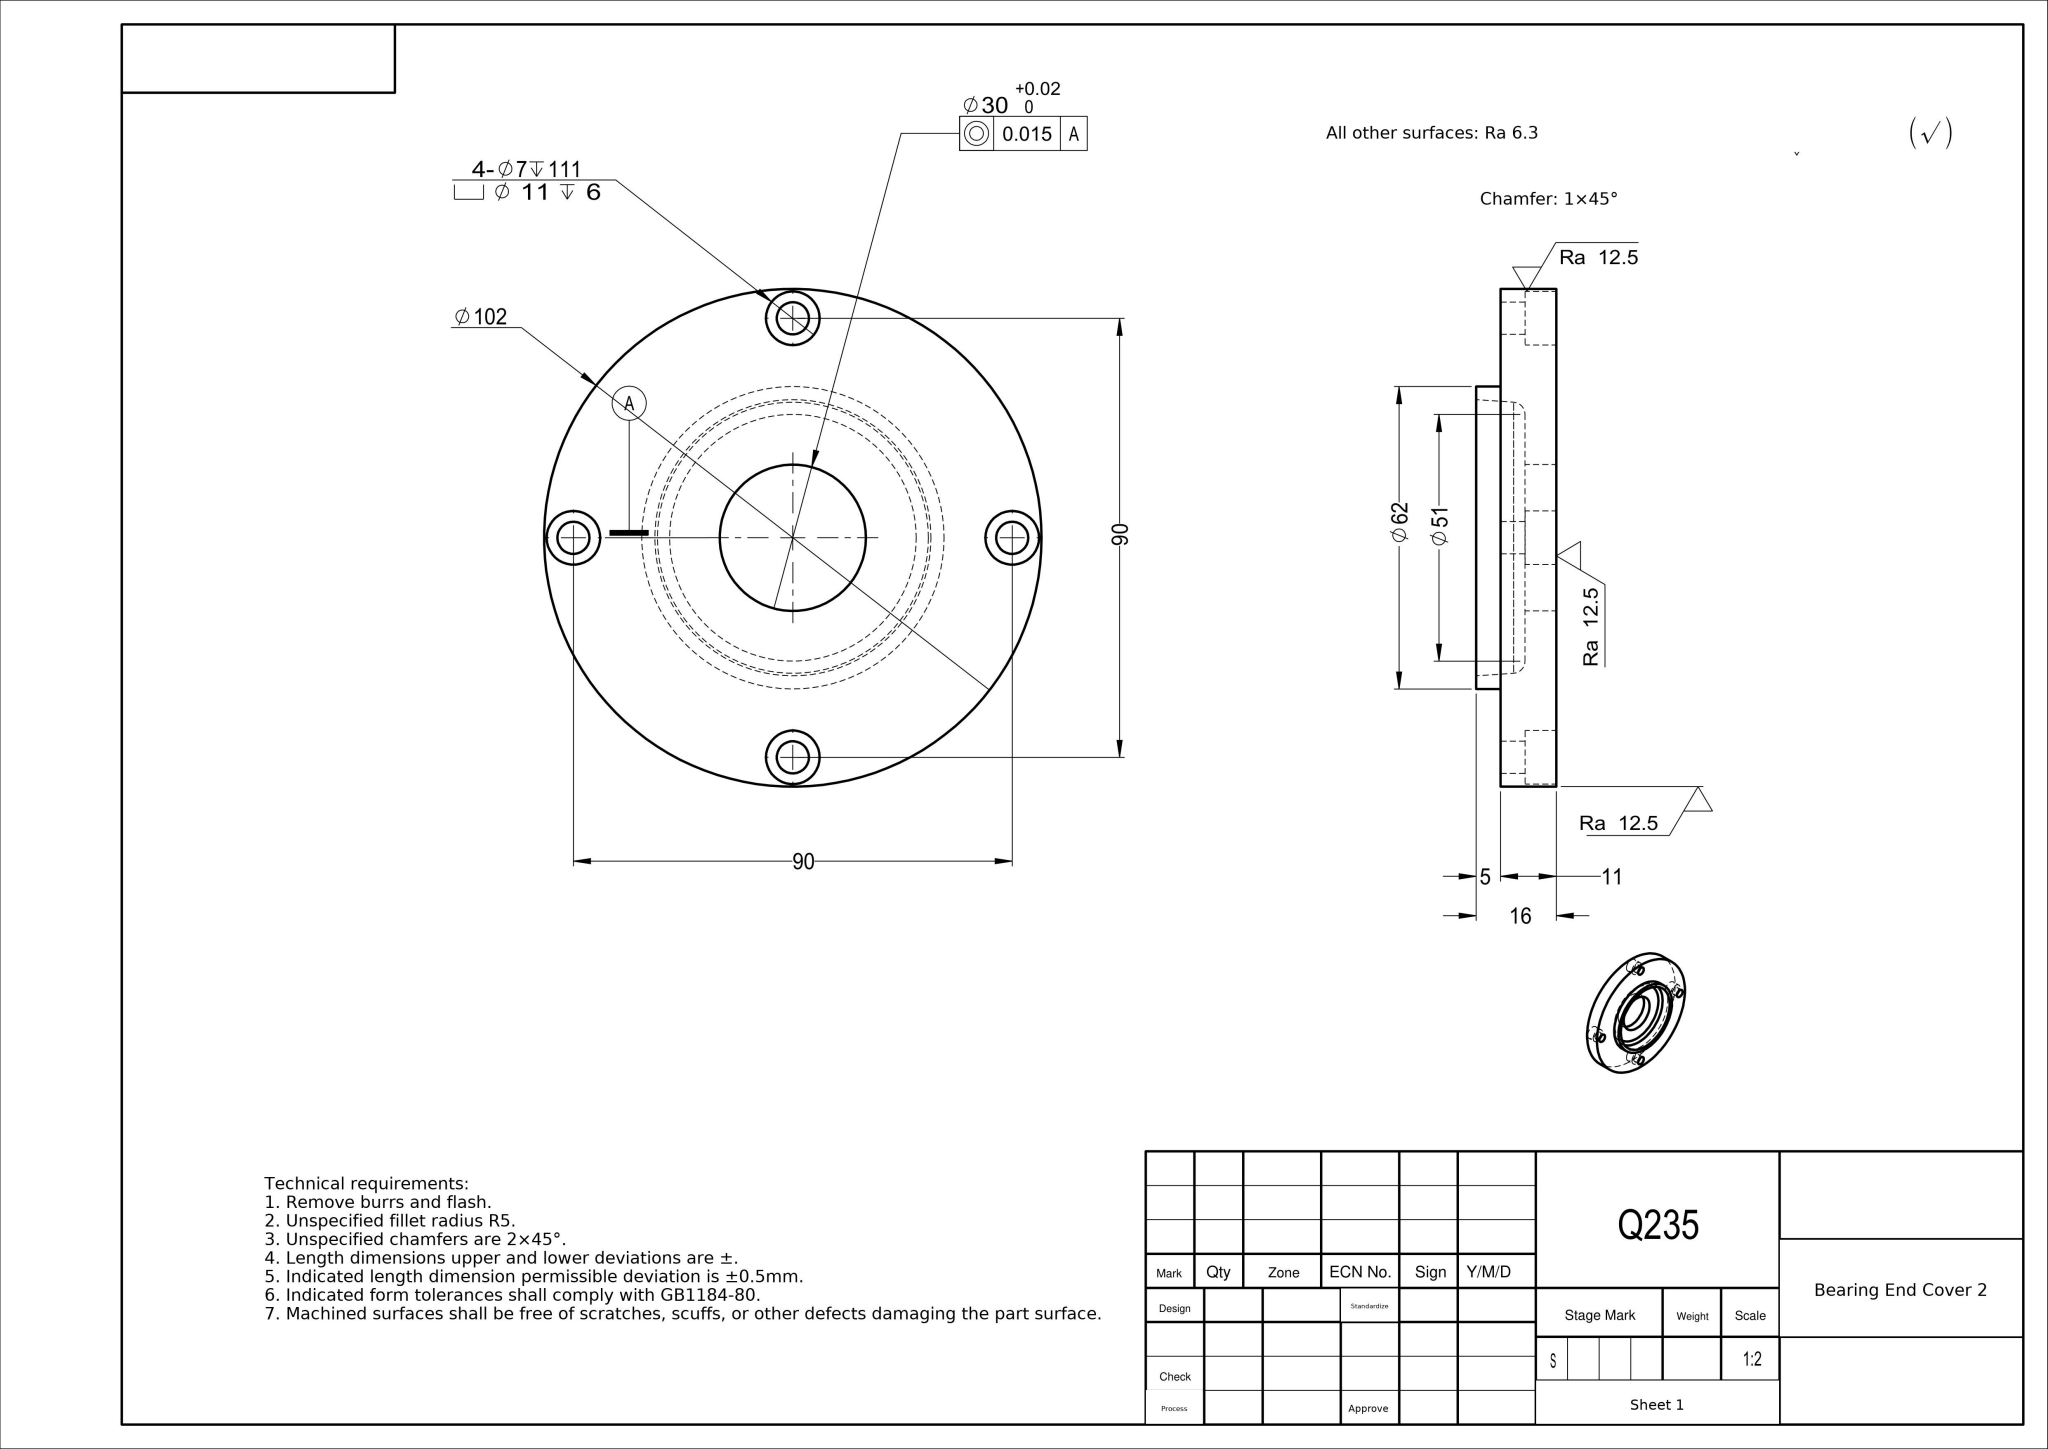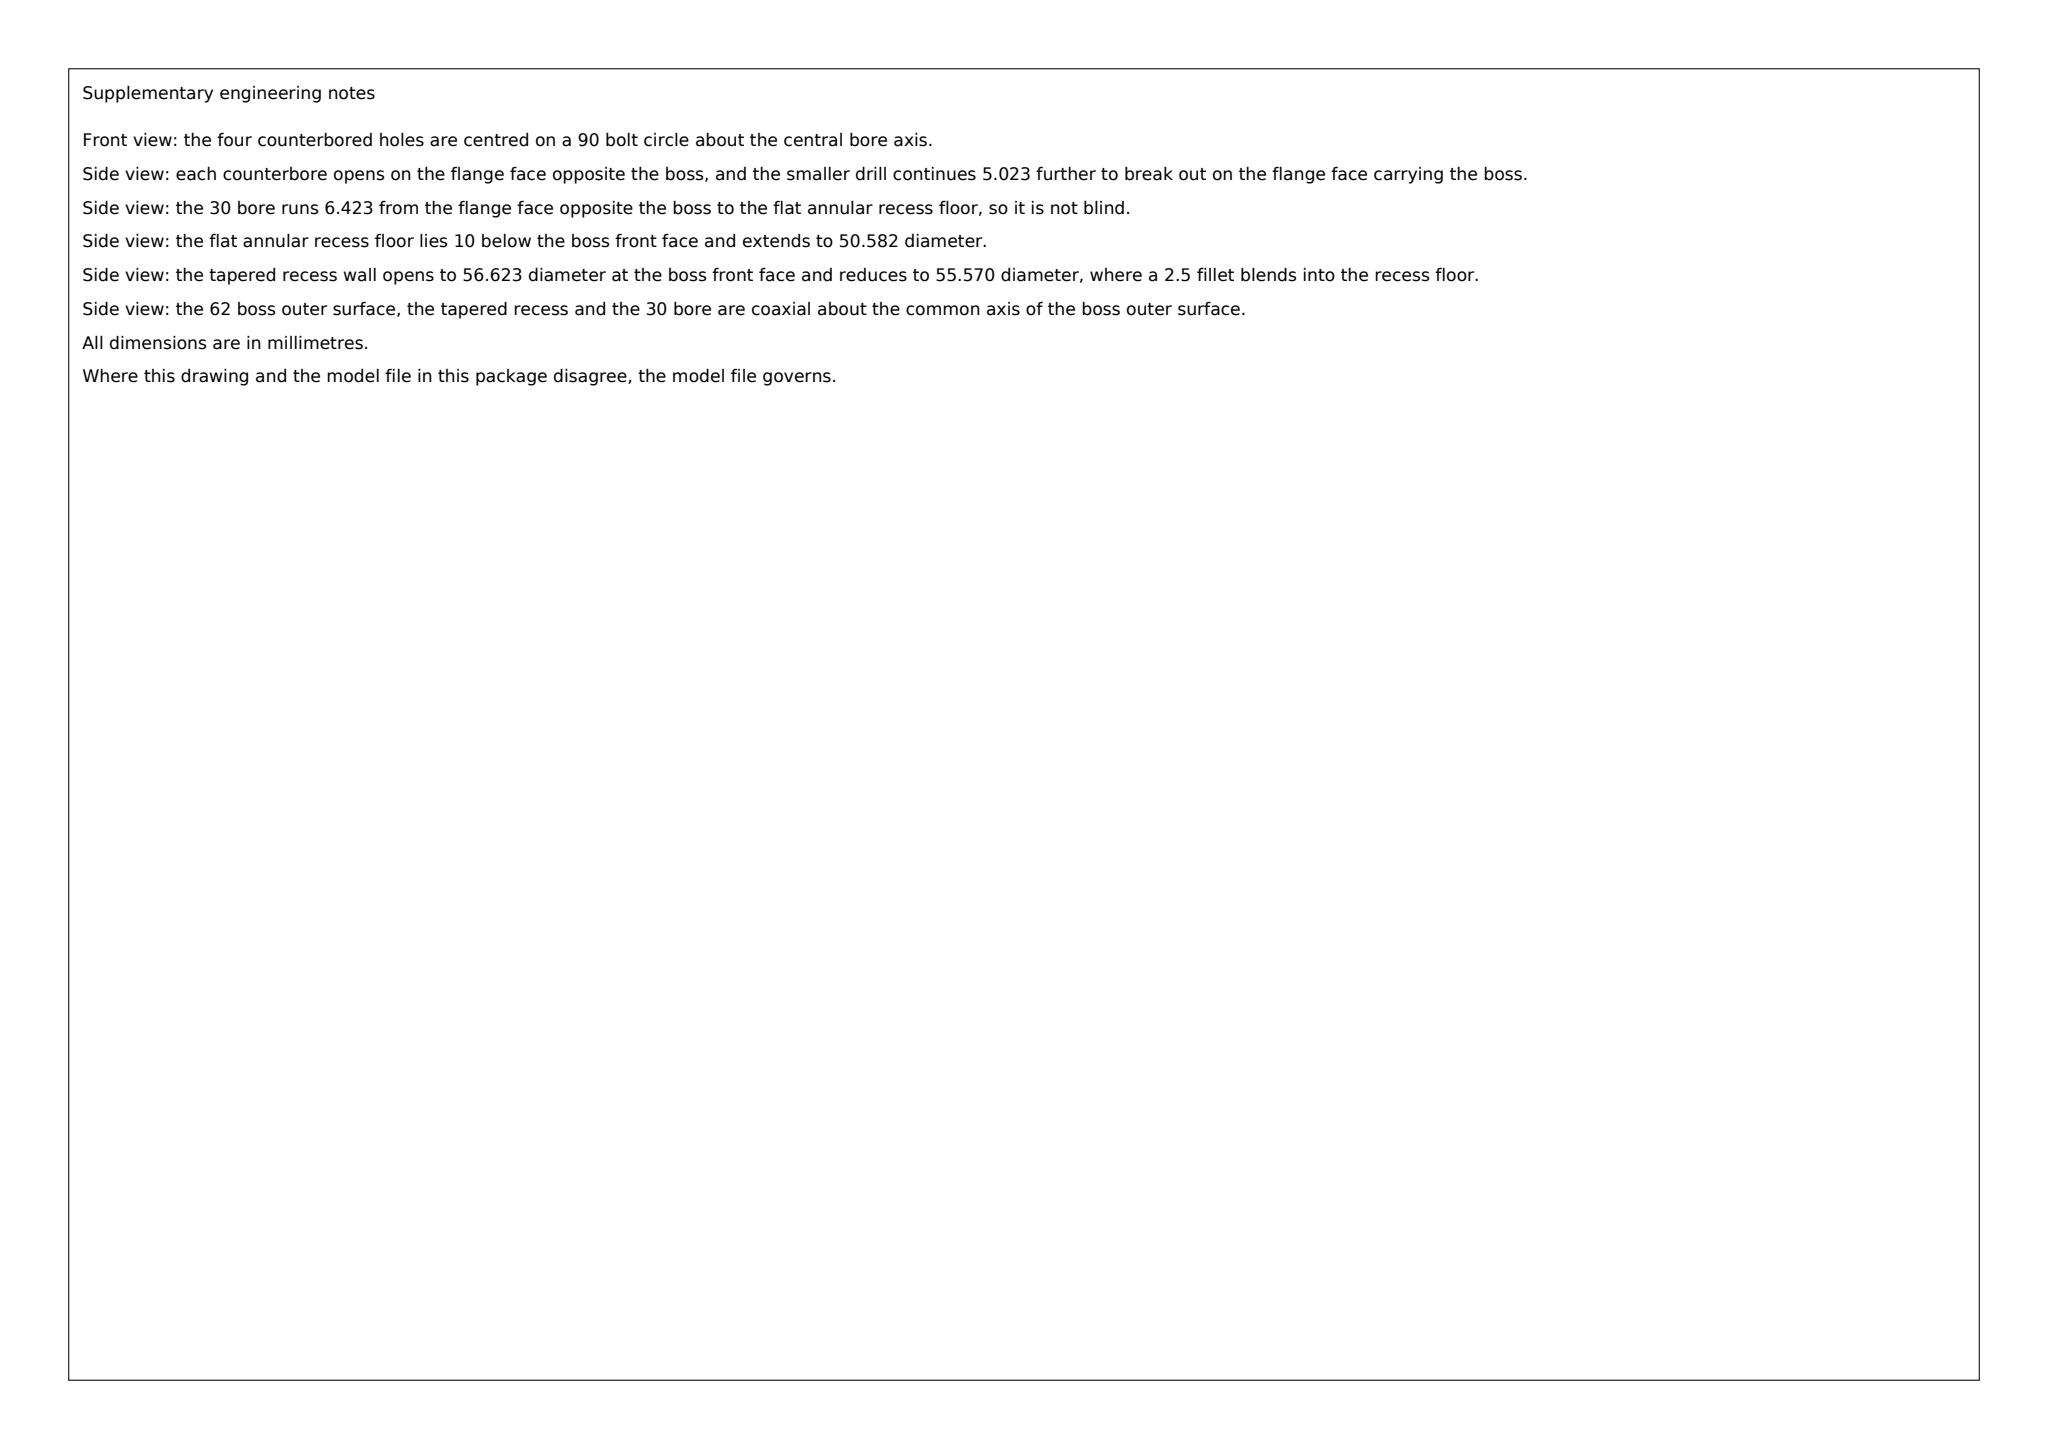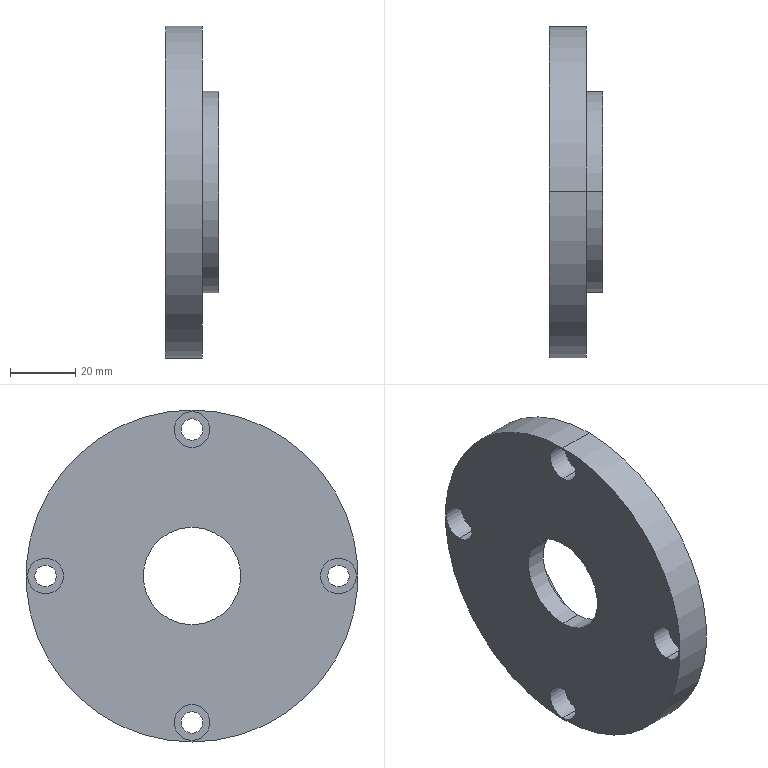Part | SolidWorks | mm | 1 solid | 34 faces | box 16.42 x 102.03 x 102.03 mm | volume 76449 mm3 | cylinder 22 | plane 8 | cone 2 | torus 2 | commonest cylinder face diameters 11 x8 6.6 x8 102.03 x2 62 x2 30 x2
Drawing notes:
4X Ø6.6 THRU (flange thickness 11.42), CBORE Ø11 DP 6.4 FROM BACK FACE (X=0 DATUM A) | from the solid: cylinders Ø6.6 L=5.02 and Ø11 L=6.4 on x axis; flange cylinder Ø102.03 L=11.42; plane x=6.4
4X Ø6.6/Ø11 CBORE HOLES EQ SP ON Ø90 BOLT CIRCLE, PATTERN CLOCKED ON THE TWO CENTERLINES (CENTERS AT ±45 FROM AXIS) | from the solid: cylinder positions (6.02,51.02),(51.02,6.02),(51.02,96.02),(96.02,51.02) about center 51.02,51.02
Ø30 +0.02/0 BORE DP 6.42 FROM COUNTERBORED FACE (X=0 DATUM A) - NOT THRU | from the solid: cylinder [30, x, (51.02,51.02), length 6.42]; plane x=6.42
INTERNAL RECESS DEPTH 10 FROM BOSS FACE (X=16.42) TO BOTTOM OF Ø30 BORE (X=6.42) | from the solid: axis_planes x=6.42 and x=16.42; bbox_x 16.423
INTERNAL TAPERED BORE 7.9° INCLUDED ANGLE, REF Ø55.57, BETWEEN X=6.42 AND BOSS FACE X=16.42 | from the solid: cones [included_angle 7.9, ref_dia 55.57]; axis_planes x=6.42, x=16.42
ALL INTERNAL FILLETS R2.5 (REPLACES GENERAL NOTE R5) | from the solid: fillet_radii [2.5, 2 instances]
BOSS Ø62 PROJECTS 5 FROM FLANGE BACK FACE (X=11.42 TO X=16.42); OVERALL LENGTH 16.42, FLANGE THICKNESS 11.42 | from the solid: cylinder [62, x, (51.02,51.02), length 5.0]; cylinder Ø102.03 L=11.42; bbox 16.423
build123d program:
from build123d import *

# Parameters (mm, degrees)
CIRPATTERN1_COUNT = 4


with BuildPart() as part:
    # Sketch1 → Revolve1 (revolve)
    with BuildSketch(Plane.XY, mode=Mode.PRIVATE) as revolve1_sk:
        with BuildLine():
            Line((362.014, 803.991), (362.014, 840.006))
            Line((362.014, 840.006), (373.437, 840.006))
            Line((373.437, 840.006), (373.437, 819.991))
            Line((373.437, 819.991), (378.437, 819.991))
            Line((378.437, 819.991), (378.437, 817.303))
            Line((378.437, 817.303), (370.765, 816.776))
            ThreePointArc((370.765, 816.776), (369.109, 815.988), (368.437, 814.282))
            Line((368.437, 814.282), (368.437, 803.991))
            Line((368.437, 803.991), (362.014, 803.991))
        make_face()
    revolve(revolve1_sk.sketch.rotate(Axis((352.045, 788.991, 0), (1, 0, 0)), 90), axis=Axis((352.045, 788.991, 0), (1, 0, 0)))

    # Sketch2 → M6 Hex Socket Head Cap Screw CBORE1 (revolve, cut)
    with BuildSketch(Plane(origin=(362.014, 833.991, 0), x_dir=(0, 0, 1), z_dir=(0, 1, 0))):
        Polygon((0, 0), (0, 112.983), (3.3, 111), (3.3, 6.4), (5.5, 6.4), (5.5, 0), align=None)
    m6_hex_socket_head_cap_screw_cbore1 = revolve(axis=Axis((355.664, 833.991, 0), (1, 0, 0)), mode=Mode.SUBTRACT)

    # CirPattern1: M6 Hex Socket Head Cap Screw CBORE1 ×4 about axis
    cirpattern1_axis = Axis((0, 788.991, 0), (1, 0, 0))
    for i in range(1, CIRPATTERN1_COUNT):
        add(m6_hex_socket_head_cap_screw_cbore1.rotate(cirpattern1_axis, i * 360 / CIRPATTERN1_COUNT), mode=Mode.SUBTRACT)


solid = part.part